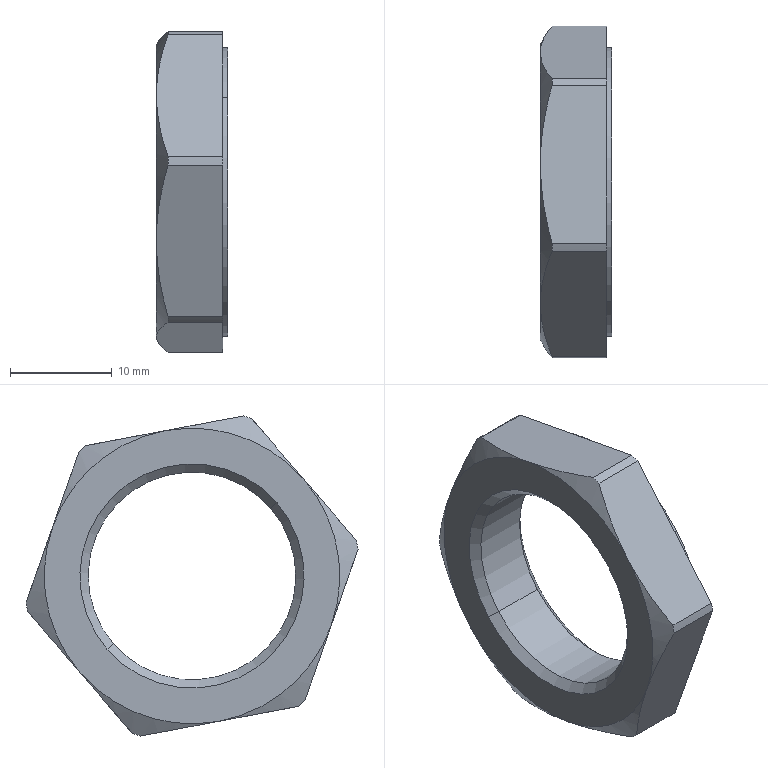Component | SolidWorks | CCDJSMA20x160SU(0)+(CS1-M-2)-1_CCDJS20 MA Nut-1 | 1 solid | 29 faces | box 7 x 32.58 x 31.42 mm | volume 2695 mm3 | cone 10 | cylinder 10 | plane 9 | commonest cylinder face diameters 33 x6 20.376 x2 28.4 x2
STEP:
#1=COLOUR_RGB('',0.7922,0.8196,0.9333);
#2=FILL_AREA_STYLE_COLOUR('',#1);
#3=FILL_AREA_STYLE('',(#2));
#4=SURFACE_STYLE_FILL_AREA(#3);
#5=SURFACE_SIDE_STYLE('',(#4));
#6=SURFACE_STYLE_USAGE(.BOTH.,#5);
#7=PRESENTATION_STYLE_ASSIGNMENT((#6));
#8=CARTESIAN_POINT('',(4.023,16.49,-2.241));
#9=VERTEX_POINT('',#8);
#10=CARTESIAN_POINT('',(4.023,17.098,-2.764));
#11=VERTEX_POINT('',#10);
#12=CARTESIAN_POINT('',(4.023,16.794,-2.503));
#13=DIRECTION('',(-1.,0.,0.));
#14=DIRECTION('',(0.,0.7584,-0.6518));
#15=AXIS2_PLACEMENT_3D('',#12,#13,#14);
#16=CIRCLE('',#15,0.4011);
#17=EDGE_CURVE('',#9,#11,#16,.T.);
#18=ORIENTED_EDGE('',*,*,#17,.T.);
#19=CARTESIAN_POINT('',(4.055,17.122,-2.785));
#20=VERTEX_POINT('',#19);
#21=CARTESIAN_POINT('',(4.055,17.122,-2.785));
#22=DIRECTION('',(0.7071,0.5363,-0.4609));
#23=VECTOR('',#22,39.37);
#24=LINE('',#21,#23);
#25=EDGE_CURVE('',#11,#20,#24,.T.);
#26=ORIENTED_EDGE('',*,*,#25,.T.);
#27=CARTESIAN_POINT('',(4.055,16.465,-2.22));
#28=VERTEX_POINT('',#27);
#29=CARTESIAN_POINT('',(4.055,16.794,-2.503));
#30=DIRECTION('',(-1.,0.,0.));
#31=DIRECTION('',(0.,0.7584,-0.6518));
#32=AXIS2_PLACEMENT_3D('',#29,#30,#31);
#33=CIRCLE('',#32,0.4331);
#34=EDGE_CURVE('',#28,#20,#33,.T.);
#35=ORIENTED_EDGE('',*,*,#34,.F.);
#36=CARTESIAN_POINT('',(4.055,16.465,-2.22));
#37=DIRECTION('',(0.7071,-0.5363,0.4609));
#38=VECTOR('',#37,39.37);
#39=LINE('',#36,#38);
#40=EDGE_CURVE('',#9,#28,#39,.T.);
#41=ORIENTED_EDGE('',*,*,#40,.F.);
#42=EDGE_LOOP('',(#18,#26,#35,#41));
#43=FACE_OUTER_BOUND('',#42,.T.);
#44=CARTESIAN_POINT('',(4.055,16.794,-2.503));
#45=DIRECTION('',(1.,0.,0.));
#46=DIRECTION('',(0.,-0.7584,0.6518));
#47=AXIS2_PLACEMENT_3D('',#44,#45,#46);
#48=CONICAL_SURFACE('',#47,0.4331,0.7854);
#49=ADVANCED_FACE('',(#43),#48,.F.);
#50=ORIENTED_EDGE('',*,*,#17,.F.);
#51=CARTESIAN_POINT('',(3.811,16.49,-2.241));
#52=VERTEX_POINT('',#51);
#53=CARTESIAN_POINT('',(4.055,16.49,-2.241));
#54=DIRECTION('',(-1.,0.,0.));
#55=VECTOR('',#54,39.37);
#56=LINE('',#53,#55);
#57=EDGE_CURVE('',#9,#52,#56,.T.);
#58=ORIENTED_EDGE('',*,*,#57,.T.);
#59=CARTESIAN_POINT('',(3.811,17.098,-2.764));
#60=VERTEX_POINT('',#59);
#61=CARTESIAN_POINT('',(3.811,16.794,-2.503));
#62=DIRECTION('',(-1.,0.,0.));
#63=DIRECTION('',(0.,0.7584,-0.6518));
#64=AXIS2_PLACEMENT_3D('',#61,#62,#63);
#65=CIRCLE('',#64,0.4011);
#66=EDGE_CURVE('',#52,#60,#65,.T.);
#67=ORIENTED_EDGE('',*,*,#66,.T.);
#68=CARTESIAN_POINT('',(4.055,17.098,-2.764));
#69=DIRECTION('',(-1.,0.,0.));
#70=VECTOR('',#69,39.37);
#71=LINE('',#68,#70);
#72=EDGE_CURVE('',#11,#60,#71,.T.);
#73=ORIENTED_EDGE('',*,*,#72,.F.);
#74=EDGE_LOOP('',(#50,#58,#67,#73));
#75=FACE_OUTER_BOUND('',#74,.T.);
#76=CARTESIAN_POINT('',(4.055,16.794,-2.503));
#77=DIRECTION('',(-1.,0.,0.));
#78=DIRECTION('',(0.,0.7584,-0.6518));
#79=AXIS2_PLACEMENT_3D('',#76,#77,#78);
#80=CYLINDRICAL_SURFACE('',#79,0.4011);
#81=ADVANCED_FACE('',(#75),#80,.F.);
#82=ORIENTED_EDGE('',*,*,#66,.F.);
#83=CARTESIAN_POINT('',(3.78,16.465,-2.22));
#84=VERTEX_POINT('',#83);
#85=CARTESIAN_POINT('',(3.811,16.49,-2.241));
#86=DIRECTION('',(-0.7071,-0.5363,0.4609));
#87=VECTOR('',#86,39.37);
#88=LINE('',#85,#87);
#89=EDGE_CURVE('',#52,#84,#88,.T.);
#90=ORIENTED_EDGE('',*,*,#89,.T.);
#91=CARTESIAN_POINT('',(3.78,17.122,-2.785));
#92=VERTEX_POINT('',#91);
#93=CARTESIAN_POINT('',(3.78,16.794,-2.503));
#94=DIRECTION('',(-1.,0.,0.));
#95=DIRECTION('',(0.,0.7584,-0.6518));
#96=AXIS2_PLACEMENT_3D('',#93,#94,#95);
#97=CIRCLE('',#96,0.4331);
#98=EDGE_CURVE('',#84,#92,#97,.T.);
#99=ORIENTED_EDGE('',*,*,#98,.T.);
#100=CARTESIAN_POINT('',(3.811,17.098,-2.764));
#101=DIRECTION('',(-0.7071,0.5363,-0.4609));
#102=VECTOR('',#101,39.37);
#103=LINE('',#100,#102);
#104=EDGE_CURVE('',#60,#92,#103,.T.);
#105=ORIENTED_EDGE('',*,*,#104,.F.);
#106=EDGE_LOOP('',(#82,#90,#99,#105));
#107=FACE_OUTER_BOUND('',#106,.T.);
#108=CARTESIAN_POINT('',(3.811,16.794,-2.503));
#109=DIRECTION('',(-1.,0.,0.));
#110=DIRECTION('',(0.,0.7584,-0.6518));
#111=AXIS2_PLACEMENT_3D('',#108,#109,#110);
#112=CONICAL_SURFACE('',#111,0.4011,0.7854);
#113=ADVANCED_FACE('',(#107),#112,.F.);
#114=CARTESIAN_POINT('',(4.055,17.218,-2.867));
#115=VERTEX_POINT('',#114);
#116=CARTESIAN_POINT('',(4.055,16.37,-2.138));
#117=VERTEX_POINT('',#116);
#118=CARTESIAN_POINT('',(4.055,16.794,-2.503));
#119=DIRECTION('',(-1.,0.,0.));
#120=DIRECTION('',(0.,0.7584,-0.6518));
#121=AXIS2_PLACEMENT_3D('',#118,#119,#120);
#122=CIRCLE('',#121,0.5591);
#123=EDGE_CURVE('',#115,#117,#122,.T.);
#124=ORIENTED_EDGE('',*,*,#123,.T.);
#125=CARTESIAN_POINT('',(4.035,16.37,-2.138));
#126=VERTEX_POINT('',#125);
#127=CARTESIAN_POINT('',(4.055,16.37,-2.138));
#128=DIRECTION('',(-1.,0.,0.));
#129=VECTOR('',#128,39.37);
#130=LINE('',#127,#129);
#131=EDGE_CURVE('',#117,#126,#130,.T.);
#132=ORIENTED_EDGE('',*,*,#131,.T.);
#133=CARTESIAN_POINT('',(4.035,17.218,-2.867));
#134=VERTEX_POINT('',#133);
#135=CARTESIAN_POINT('',(4.035,16.794,-2.503));
#136=DIRECTION('',(-1.,0.,0.));
#137=DIRECTION('',(0.,0.7584,-0.6518));
#138=AXIS2_PLACEMENT_3D('',#135,#136,#137);
#139=CIRCLE('',#138,0.5591);
#140=EDGE_CURVE('',#134,#126,#139,.T.);
#141=ORIENTED_EDGE('',*,*,#140,.F.);
#142=CARTESIAN_POINT('',(4.055,17.218,-2.867));
#143=DIRECTION('',(-1.,0.,0.));
#144=VECTOR('',#143,39.37);
#145=LINE('',#142,#144);
#146=EDGE_CURVE('',#115,#134,#145,.T.);
#147=ORIENTED_EDGE('',*,*,#146,.F.);
#148=EDGE_LOOP('',(#124,#132,#141,#147));
#149=FACE_OUTER_BOUND('',#148,.T.);
#150=CARTESIAN_POINT('',(4.055,16.794,-2.503));
#151=DIRECTION('',(-1.,0.,0.));
#152=DIRECTION('',(0.,0.7584,-0.6518));
#153=AXIS2_PLACEMENT_3D('',#150,#151,#152);
#154=CYLINDRICAL_SURFACE('',#153,0.5591);
#155=ADVANCED_FACE('',(#149),#154,.T.);
#156=CARTESIAN_POINT('',(3.825,17.435,-2.606));
#157=VERTEX_POINT('',#156);
#158=CARTESIAN_POINT('',(3.825,17.429,-2.64));
#159=VERTEX_POINT('',#158);
#160=CARTESIAN_POINT('',(3.825,16.794,-2.503));
#161=DIRECTION('',(-1.,0.,0.));
#162=DIRECTION('',(0.,0.7584,-0.6518));
#163=AXIS2_PLACEMENT_3D('',#160,#161,#162);
#164=CIRCLE('',#163,0.6496);
#165=EDGE_CURVE('',#157,#159,#164,.T.);
#166=ORIENTED_EDGE('',*,*,#165,.T.);
#167=CARTESIAN_POINT('',(3.78,17.227,-2.875));
#168=VERTEX_POINT('',#167);
#169=CARTESIAN_POINT('',(3.825,17.429,-2.64));
#170=CARTESIAN_POINT('',(3.811,17.396,-2.678));
#171=CARTESIAN_POINT('',(3.799,17.362,-2.717));
#172=CARTESIAN_POINT('',(3.784,17.295,-2.796));
#173=CARTESIAN_POINT('',(3.78,17.261,-2.835));
#174=CARTESIAN_POINT('',(3.78,17.227,-2.875));
#175=B_SPLINE_CURVE_WITH_KNOTS('',3,(#169,#170,#171,#172,#173,#174),.UNSPECIFIED.,.F.,.F.,(4,2,4),(0.01543,0.01941,0.02338),.UNSPECIFIED.);
#176=EDGE_CURVE('',#159,#168,#175,.T.);
#177=ORIENTED_EDGE('',*,*,#176,.T.);
#178=CARTESIAN_POINT('',(3.78,17.333,-2.314));
#179=VERTEX_POINT('',#178);
#180=CARTESIAN_POINT('',(3.78,16.794,-2.503));
#181=DIRECTION('',(-1.,0.,0.));
#182=DIRECTION('',(0.,0.7584,-0.6518));
#183=AXIS2_PLACEMENT_3D('',#180,#181,#182);
#184=CIRCLE('',#183,0.5709);
#185=EDGE_CURVE('',#179,#168,#184,.T.);
#186=ORIENTED_EDGE('',*,*,#185,.F.);
#187=CARTESIAN_POINT('',(3.78,17.333,-2.314));
#188=CARTESIAN_POINT('',(3.78,17.341,-2.339));
#189=CARTESIAN_POINT('',(3.781,17.35,-2.363));
#190=CARTESIAN_POINT('',(3.785,17.367,-2.413));
#191=CARTESIAN_POINT('',(3.788,17.376,-2.437));
#192=CARTESIAN_POINT('',(3.8,17.401,-2.51));
#193=CARTESIAN_POINT('',(3.811,17.418,-2.559));
#194=CARTESIAN_POINT('',(3.825,17.435,-2.606));
#195=B_SPLINE_CURVE_WITH_KNOTS('',3,(#187,#188,#189,#190,#191,#192,#193,#194),.UNSPECIFIED.,.F.,.F.,(4,2,2,4),(0.007958,0.009936,0.01191,0.01587),.UNSPECIFIED.);
#196=EDGE_CURVE('',#179,#157,#195,.T.);
#197=ORIENTED_EDGE('',*,*,#196,.T.);
#198=EDGE_LOOP('',(#166,#177,#186,#197));
#199=FACE_OUTER_BOUND('',#198,.T.);
#200=CARTESIAN_POINT('',(3.825,16.794,-2.503));
#201=DIRECTION('',(1.,0.,0.));
#202=DIRECTION('',(0.,-0.7584,0.6518));
#203=AXIS2_PLACEMENT_3D('',#200,#201,#202);
#204=CONICAL_SURFACE('',#203,0.6496,1.047);
#205=ADVANCED_FACE('',(#199),#204,.T.);
#206=CARTESIAN_POINT('',(3.825,17.204,-1.999));
#207=VERTEX_POINT('',#206);
#208=CARTESIAN_POINT('',(3.825,17.23,-2.021));
#209=VERTEX_POINT('',#208);
#210=CARTESIAN_POINT('',(3.825,16.794,-2.503));
#211=DIRECTION('',(-1.,0.,0.));
#212=DIRECTION('',(0.,0.7584,-0.6518));
#213=AXIS2_PLACEMENT_3D('',#210,#211,#212);
#214=CIRCLE('',#213,0.6496);
#215=EDGE_CURVE('',#207,#209,#214,.T.);
#216=ORIENTED_EDGE('',*,*,#215,.T.);
#217=CARTESIAN_POINT('',(3.825,17.23,-2.021));
#218=CARTESIAN_POINT('',(3.811,17.247,-2.069));
#219=CARTESIAN_POINT('',(3.8,17.264,-2.118));
#220=CARTESIAN_POINT('',(3.784,17.298,-2.215));
#221=CARTESIAN_POINT('',(3.78,17.315,-2.264));
#222=CARTESIAN_POINT('',(3.78,17.333,-2.314));
#223=B_SPLINE_CURVE_WITH_KNOTS('',3,(#217,#218,#219,#220,#221,#222),.UNSPECIFIED.,.F.,.F.,(4,2,4),(0.00000075,0.003979,0.007958),.UNSPECIFIED.);
#224=EDGE_CURVE('',#209,#179,#223,.T.);
#225=ORIENTED_EDGE('',*,*,#224,.T.);
#226=CARTESIAN_POINT('',(3.78,16.9,-1.942));
#227=VERTEX_POINT('',#226);
#228=CARTESIAN_POINT('',(3.78,16.794,-2.503));
#229=DIRECTION('',(-1.,0.,0.));
#230=DIRECTION('',(0.,0.7584,-0.6518));
#231=AXIS2_PLACEMENT_3D('',#228,#229,#230);
#232=CIRCLE('',#231,0.5709);
#233=EDGE_CURVE('',#227,#179,#232,.T.);
#234=ORIENTED_EDGE('',*,*,#233,.F.);
#235=CARTESIAN_POINT('',(3.78,16.9,-1.942));
#236=CARTESIAN_POINT('',(3.78,16.925,-1.947));
#237=CARTESIAN_POINT('',(3.781,16.951,-1.952));
#238=CARTESIAN_POINT('',(3.785,17.003,-1.961));
#239=CARTESIAN_POINT('',(3.788,17.028,-1.966));
#240=CARTESIAN_POINT('',(3.8,17.104,-1.98));
#241=CARTESIAN_POINT('',(3.811,17.155,-1.99));
#242=CARTESIAN_POINT('',(3.825,17.204,-1.999));
#243=B_SPLINE_CURVE_WITH_KNOTS('',3,(#235,#236,#237,#238,#239,#240,#241,#242),.UNSPECIFIED.,.F.,.F.,(4,2,2,4),(0.007958,0.009936,0.01191,0.01587),.UNSPECIFIED.);
#244=EDGE_CURVE('',#227,#207,#243,.T.);
#245=ORIENTED_EDGE('',*,*,#244,.T.);
#246=EDGE_LOOP('',(#216,#225,#234,#245));
#247=FACE_OUTER_BOUND('',#246,.T.);
#248=CARTESIAN_POINT('',(3.825,16.794,-2.503));
#249=DIRECTION('',(1.,0.,0.));
#250=DIRECTION('',(0.,-0.7584,0.6518));
#251=AXIS2_PLACEMENT_3D('',#248,#249,#250);
#252=CONICAL_SURFACE('',#251,0.6496,1.047);
#253=ADVANCED_FACE('',(#247),#252,.T.);
#254=CARTESIAN_POINT('',(3.825,16.563,-1.896));
#255=VERTEX_POINT('',#254);
#256=CARTESIAN_POINT('',(3.825,16.595,-1.884));
#257=VERTEX_POINT('',#256);
#258=CARTESIAN_POINT('',(3.825,16.794,-2.503));
#259=DIRECTION('',(-1.,0.,0.));
#260=DIRECTION('',(0.,0.7584,-0.6518));
#261=AXIS2_PLACEMENT_3D('',#258,#259,#260);
#262=CIRCLE('',#261,0.6496);
#263=EDGE_CURVE('',#255,#257,#262,.T.);
#264=ORIENTED_EDGE('',*,*,#263,.T.);
#265=CARTESIAN_POINT('',(3.825,16.595,-1.884));
#266=CARTESIAN_POINT('',(3.811,16.645,-1.894));
#267=CARTESIAN_POINT('',(3.8,16.695,-1.903));
#268=CARTESIAN_POINT('',(3.784,16.797,-1.922));
#269=CARTESIAN_POINT('',(3.78,16.848,-1.932));
#270=CARTESIAN_POINT('',(3.78,16.9,-1.942));
#271=B_SPLINE_CURVE_WITH_KNOTS('',3,(#265,#266,#267,#268,#269,#270),.UNSPECIFIED.,.F.,.F.,(4,2,4),(0.00000075,0.003979,0.007958),.UNSPECIFIED.);
#272=EDGE_CURVE('',#257,#227,#271,.T.);
#273=ORIENTED_EDGE('',*,*,#272,.T.);
#274=CARTESIAN_POINT('',(3.78,16.361,-2.131));
#275=VERTEX_POINT('',#274);
#276=CARTESIAN_POINT('',(3.78,16.794,-2.503));
#277=DIRECTION('',(-1.,0.,0.));
#278=DIRECTION('',(0.,0.7584,-0.6518));
#279=AXIS2_PLACEMENT_3D('',#276,#277,#278);
#280=CIRCLE('',#279,0.5709);
#281=EDGE_CURVE('',#275,#227,#280,.T.);
#282=ORIENTED_EDGE('',*,*,#281,.F.);
#283=CARTESIAN_POINT('',(3.78,16.361,-2.131));
#284=CARTESIAN_POINT('',(3.78,16.395,-2.091));
#285=CARTESIAN_POINT('',(3.784,16.429,-2.052));
#286=CARTESIAN_POINT('',(3.799,16.496,-1.973));
#287=CARTESIAN_POINT('',(3.811,16.53,-1.934));
#288=CARTESIAN_POINT('',(3.825,16.563,-1.896));
#289=B_SPLINE_CURVE_WITH_KNOTS('',3,(#283,#284,#285,#286,#287,#288),.UNSPECIFIED.,.F.,.F.,(4,2,4),(0.01461,0.01858,0.02255),.UNSPECIFIED.);
#290=EDGE_CURVE('',#275,#255,#289,.T.);
#291=ORIENTED_EDGE('',*,*,#290,.T.);
#292=EDGE_LOOP('',(#264,#273,#282,#291));
#293=FACE_OUTER_BOUND('',#292,.T.);
#294=CARTESIAN_POINT('',(3.825,16.794,-2.503));
#295=DIRECTION('',(1.,0.,0.));
#296=DIRECTION('',(0.,-0.7584,0.6518));
#297=AXIS2_PLACEMENT_3D('',#294,#295,#296);
#298=CONICAL_SURFACE('',#297,0.6496,1.047);
#299=ADVANCED_FACE('',(#293),#298,.T.);
#300=CARTESIAN_POINT('',(3.825,16.153,-2.399));
#301=VERTEX_POINT('',#300);
#302=CARTESIAN_POINT('',(3.825,16.159,-2.366));
#303=VERTEX_POINT('',#302);
#304=CARTESIAN_POINT('',(3.825,16.794,-2.503));
#305=DIRECTION('',(-1.,0.,0.));
#306=DIRECTION('',(0.,0.7584,-0.6518));
#307=AXIS2_PLACEMENT_3D('',#304,#305,#306);
#308=CIRCLE('',#307,0.6496);
#309=EDGE_CURVE('',#301,#303,#308,.T.);
#310=ORIENTED_EDGE('',*,*,#309,.T.);
#311=CARTESIAN_POINT('',(3.825,16.159,-2.366));
#312=CARTESIAN_POINT('',(3.811,16.192,-2.328));
#313=CARTESIAN_POINT('',(3.8,16.225,-2.289));
#314=CARTESIAN_POINT('',(3.788,16.275,-2.23));
#315=CARTESIAN_POINT('',(3.785,16.292,-2.21));
#316=CARTESIAN_POINT('',(3.781,16.327,-2.17));
#317=CARTESIAN_POINT('',(3.78,16.344,-2.151));
#318=CARTESIAN_POINT('',(3.78,16.361,-2.131));
#319=B_SPLINE_CURVE_WITH_KNOTS('',3,(#311,#312,#313,#314,#315,#316,#317,#318),.UNSPECIFIED.,.F.,.F.,(4,2,2,4),(0.006677,0.01064,0.01263,0.01461),.UNSPECIFIED.);
#320=EDGE_CURVE('',#303,#275,#319,.T.);
#321=ORIENTED_EDGE('',*,*,#320,.T.);
#322=CARTESIAN_POINT('',(3.78,16.255,-2.692));
#323=VERTEX_POINT('',#322);
#324=CARTESIAN_POINT('',(3.78,16.794,-2.503));
#325=DIRECTION('',(-1.,0.,0.));
#326=DIRECTION('',(0.,0.7584,-0.6518));
#327=AXIS2_PLACEMENT_3D('',#324,#325,#326);
#328=CIRCLE('',#327,0.5709);
#329=EDGE_CURVE('',#323,#275,#328,.T.);
#330=ORIENTED_EDGE('',*,*,#329,.F.);
#331=CARTESIAN_POINT('',(3.78,16.255,-2.692));
#332=CARTESIAN_POINT('',(3.78,16.247,-2.667));
#333=CARTESIAN_POINT('',(3.781,16.238,-2.642));
#334=CARTESIAN_POINT('',(3.785,16.22,-2.593));
#335=CARTESIAN_POINT('',(3.788,16.212,-2.568));
#336=CARTESIAN_POINT('',(3.8,16.186,-2.495));
#337=CARTESIAN_POINT('',(3.811,16.169,-2.447));
#338=CARTESIAN_POINT('',(3.825,16.153,-2.399));
#339=B_SPLINE_CURVE_WITH_KNOTS('',3,(#331,#332,#333,#334,#335,#336,#337,#338),.UNSPECIFIED.,.F.,.F.,(4,2,2,4),(0.007958,0.009936,0.01191,0.01587),.UNSPECIFIED.);
#340=EDGE_CURVE('',#323,#301,#339,.T.);
#341=ORIENTED_EDGE('',*,*,#340,.T.);
#342=EDGE_LOOP('',(#310,#321,#330,#341));
#343=FACE_OUTER_BOUND('',#342,.T.);
#344=CARTESIAN_POINT('',(3.825,16.794,-2.503));
#345=DIRECTION('',(1.,0.,0.));
#346=DIRECTION('',(0.,-0.7584,0.6518));
#347=AXIS2_PLACEMENT_3D('',#344,#345,#346);
#348=CONICAL_SURFACE('',#347,0.6496,1.047);
#349=ADVANCED_FACE('',(#343),#348,.T.);
#350=CARTESIAN_POINT('',(3.825,16.383,-3.006));
#351=VERTEX_POINT('',#350);
#352=CARTESIAN_POINT('',(3.825,16.358,-2.984));
#353=VERTEX_POINT('',#352);
#354=CARTESIAN_POINT('',(3.825,16.794,-2.503));
#355=DIRECTION('',(-1.,0.,0.));
#356=DIRECTION('',(0.,0.7584,-0.6518));
#357=AXIS2_PLACEMENT_3D('',#354,#355,#356);
#358=CIRCLE('',#357,0.6496);
#359=EDGE_CURVE('',#351,#353,#358,.T.);
#360=ORIENTED_EDGE('',*,*,#359,.T.);
#361=CARTESIAN_POINT('',(3.825,16.358,-2.984));
#362=CARTESIAN_POINT('',(3.811,16.341,-2.936));
#363=CARTESIAN_POINT('',(3.8,16.324,-2.888));
#364=CARTESIAN_POINT('',(3.784,16.29,-2.79));
#365=CARTESIAN_POINT('',(3.78,16.273,-2.741));
#366=CARTESIAN_POINT('',(3.78,16.255,-2.692));
#367=B_SPLINE_CURVE_WITH_KNOTS('',3,(#361,#362,#363,#364,#365,#366),.UNSPECIFIED.,.F.,.F.,(4,2,4),(0.00000075,0.003979,0.007958),.UNSPECIFIED.);
#368=EDGE_CURVE('',#353,#323,#367,.T.);
#369=ORIENTED_EDGE('',*,*,#368,.T.);
#370=CARTESIAN_POINT('',(3.78,16.688,-3.064));
#371=VERTEX_POINT('',#370);
#372=CARTESIAN_POINT('',(3.78,16.794,-2.503));
#373=DIRECTION('',(-1.,0.,0.));
#374=DIRECTION('',(0.,0.7584,-0.6518));
#375=AXIS2_PLACEMENT_3D('',#372,#373,#374);
#376=CIRCLE('',#375,0.5709);
#377=EDGE_CURVE('',#371,#323,#376,.T.);
#378=ORIENTED_EDGE('',*,*,#377,.F.);
#379=CARTESIAN_POINT('',(3.78,16.688,-3.064));
#380=CARTESIAN_POINT('',(3.78,16.662,-3.059));
#381=CARTESIAN_POINT('',(3.781,16.636,-3.054));
#382=CARTESIAN_POINT('',(3.785,16.585,-3.044));
#383=CARTESIAN_POINT('',(3.788,16.56,-3.04));
#384=CARTESIAN_POINT('',(3.8,16.483,-3.025));
#385=CARTESIAN_POINT('',(3.811,16.433,-3.016));
#386=CARTESIAN_POINT('',(3.825,16.383,-3.006));
#387=B_SPLINE_CURVE_WITH_KNOTS('',3,(#379,#380,#381,#382,#383,#384,#385,#386),.UNSPECIFIED.,.F.,.F.,(4,2,2,4),(0.007958,0.009936,0.01191,0.01587),.UNSPECIFIED.);
#388=EDGE_CURVE('',#371,#351,#387,.T.);
#389=ORIENTED_EDGE('',*,*,#388,.T.);
#390=EDGE_LOOP('',(#360,#369,#378,#389));
#391=FACE_OUTER_BOUND('',#390,.T.);
#392=CARTESIAN_POINT('',(3.825,16.794,-2.503));
#393=DIRECTION('',(1.,0.,0.));
#394=DIRECTION('',(0.,-0.7584,0.6518));
#395=AXIS2_PLACEMENT_3D('',#392,#393,#394);
#396=CONICAL_SURFACE('',#395,0.6496,1.047);
#397=ADVANCED_FACE('',(#391),#396,.T.);
#398=CARTESIAN_POINT('',(4.035,17.435,-2.606));
#399=VERTEX_POINT('',#398);
#400=CARTESIAN_POINT('',(4.035,17.429,-2.64));
#401=VERTEX_POINT('',#400);
#402=CARTESIAN_POINT('',(4.035,16.794,-2.503));
#403=DIRECTION('',(-1.,0.,0.));
#404=DIRECTION('',(0.,0.7584,-0.6518));
#405=AXIS2_PLACEMENT_3D('',#402,#403,#404);
#406=CIRCLE('',#405,0.6496);
#407=EDGE_CURVE('',#399,#401,#406,.T.);
#408=ORIENTED_EDGE('',*,*,#407,.T.);
#409=CARTESIAN_POINT('',(4.055,17.429,-2.64));
#410=DIRECTION('',(-1.,0.,0.));
#411=VECTOR('',#410,39.37);
#412=LINE('',#409,#411);
#413=EDGE_CURVE('',#401,#159,#412,.T.);
#414=ORIENTED_EDGE('',*,*,#413,.T.);
#415=ORIENTED_EDGE('',*,*,#165,.F.);
#416=CARTESIAN_POINT('',(4.055,17.435,-2.606));
#417=DIRECTION('',(1.,0.,0.));
#418=VECTOR('',#417,39.37);
#419=LINE('',#416,#418);
#420=EDGE_CURVE('',#157,#399,#419,.T.);
#421=ORIENTED_EDGE('',*,*,#420,.T.);
#422=EDGE_LOOP('',(#408,#414,#415,#421));
#423=FACE_OUTER_BOUND('',#422,.T.);
#424=CARTESIAN_POINT('',(4.055,16.794,-2.503));
#425=DIRECTION('',(-1.,0.,0.));
#426=DIRECTION('',(0.,0.7584,-0.6518));
#427=AXIS2_PLACEMENT_3D('',#424,#425,#426);
#428=CYLINDRICAL_SURFACE('',#427,0.6496);
#429=ADVANCED_FACE('',(#423),#428,.T.);
#430=CARTESIAN_POINT('',(4.035,17.204,-1.999));
#431=VERTEX_POINT('',#430);
#432=CARTESIAN_POINT('',(4.035,17.23,-2.021));
#433=VERTEX_POINT('',#432);
#434=CARTESIAN_POINT('',(4.035,16.794,-2.503));
#435=DIRECTION('',(-1.,0.,0.));
#436=DIRECTION('',(0.,0.7584,-0.6518));
#437=AXIS2_PLACEMENT_3D('',#434,#435,#436);
#438=CIRCLE('',#437,0.6496);
#439=EDGE_CURVE('',#431,#433,#438,.T.);
#440=ORIENTED_EDGE('',*,*,#439,.T.);
#441=CARTESIAN_POINT('',(4.055,17.23,-2.021));
#442=DIRECTION('',(-1.,0.,0.));
#443=VECTOR('',#442,39.37);
#444=LINE('',#441,#443);
#445=EDGE_CURVE('',#433,#209,#444,.T.);
#446=ORIENTED_EDGE('',*,*,#445,.T.);
#447=ORIENTED_EDGE('',*,*,#215,.F.);
#448=CARTESIAN_POINT('',(4.055,17.204,-1.999));
#449=DIRECTION('',(1.,0.,0.));
#450=VECTOR('',#449,39.37);
#451=LINE('',#448,#450);
#452=EDGE_CURVE('',#207,#431,#451,.T.);
#453=ORIENTED_EDGE('',*,*,#452,.T.);
#454=EDGE_LOOP('',(#440,#446,#447,#453));
#455=FACE_OUTER_BOUND('',#454,.T.);
#456=CARTESIAN_POINT('',(4.055,16.794,-2.503));
#457=DIRECTION('',(-1.,0.,0.));
#458=DIRECTION('',(0.,0.7584,-0.6518));
#459=AXIS2_PLACEMENT_3D('',#456,#457,#458);
#460=CYLINDRICAL_SURFACE('',#459,0.6496);
#461=ADVANCED_FACE('',(#455),#460,.T.);
#462=CARTESIAN_POINT('',(4.035,16.563,-1.896));
#463=VERTEX_POINT('',#462);
#464=CARTESIAN_POINT('',(4.035,16.595,-1.884));
#465=VERTEX_POINT('',#464);
#466=CARTESIAN_POINT('',(4.035,16.794,-2.503));
#467=DIRECTION('',(-1.,0.,0.));
#468=DIRECTION('',(0.,0.7584,-0.6518));
#469=AXIS2_PLACEMENT_3D('',#466,#467,#468);
#470=CIRCLE('',#469,0.6496);
#471=EDGE_CURVE('',#463,#465,#470,.T.);
#472=ORIENTED_EDGE('',*,*,#471,.T.);
#473=CARTESIAN_POINT('',(4.055,16.595,-1.884));
#474=DIRECTION('',(-1.,0.,0.));
#475=VECTOR('',#474,39.37);
#476=LINE('',#473,#475);
#477=EDGE_CURVE('',#465,#257,#476,.T.);
#478=ORIENTED_EDGE('',*,*,#477,.T.);
#479=ORIENTED_EDGE('',*,*,#263,.F.);
#480=CARTESIAN_POINT('',(4.055,16.563,-1.896));
#481=DIRECTION('',(1.,0.,0.));
#482=VECTOR('',#481,39.37);
#483=LINE('',#480,#482);
#484=EDGE_CURVE('',#255,#463,#483,.T.);
#485=ORIENTED_EDGE('',*,*,#484,.T.);
#486=EDGE_LOOP('',(#472,#478,#479,#485));
#487=FACE_OUTER_BOUND('',#486,.T.);
#488=CARTESIAN_POINT('',(4.055,16.794,-2.503));
#489=DIRECTION('',(-1.,0.,0.));
#490=DIRECTION('',(0.,0.7584,-0.6518));
#491=AXIS2_PLACEMENT_3D('',#488,#489,#490);
#492=CYLINDRICAL_SURFACE('',#491,0.6496);
#493=ADVANCED_FACE('',(#487),#492,.T.);
#494=CARTESIAN_POINT('',(4.035,16.153,-2.399));
#495=VERTEX_POINT('',#494);
#496=CARTESIAN_POINT('',(4.035,16.159,-2.366));
#497=VERTEX_POINT('',#496);
#498=CARTESIAN_POINT('',(4.035,16.794,-2.503));
#499=DIRECTION('',(-1.,0.,0.));
#500=DIRECTION('',(0.,0.7584,-0.6518));
#501=AXIS2_PLACEMENT_3D('',#498,#499,#500);
#502=CIRCLE('',#501,0.6496);
#503=EDGE_CURVE('',#495,#497,#502,.T.);
#504=ORIENTED_EDGE('',*,*,#503,.T.);
#505=CARTESIAN_POINT('',(4.055,16.159,-2.366));
#506=DIRECTION('',(-1.,0.,0.));
#507=VECTOR('',#506,39.37);
#508=LINE('',#505,#507);
#509=EDGE_CURVE('',#497,#303,#508,.T.);
#510=ORIENTED_EDGE('',*,*,#509,.T.);
#511=ORIENTED_EDGE('',*,*,#309,.F.);
#512=CARTESIAN_POINT('',(4.055,16.153,-2.399));
#513=DIRECTION('',(1.,0.,0.));
#514=VECTOR('',#513,39.37);
#515=LINE('',#512,#514);
#516=EDGE_CURVE('',#301,#495,#515,.T.);
#517=ORIENTED_EDGE('',*,*,#516,.T.);
#518=EDGE_LOOP('',(#504,#510,#511,#517));
#519=FACE_OUTER_BOUND('',#518,.T.);
#520=CARTESIAN_POINT('',(4.055,16.794,-2.503));
#521=DIRECTION('',(-1.,0.,0.));
#522=DIRECTION('',(0.,0.7584,-0.6518));
#523=AXIS2_PLACEMENT_3D('',#520,#521,#522);
#524=CYLINDRICAL_SURFACE('',#523,0.6496);
#525=ADVANCED_FACE('',(#519),#524,.T.);
#526=CARTESIAN_POINT('',(4.035,16.383,-3.006));
#527=VERTEX_POINT('',#526);
#528=CARTESIAN_POINT('',(4.035,16.358,-2.984));
#529=VERTEX_POINT('',#528);
#530=CARTESIAN_POINT('',(4.035,16.794,-2.503));
#531=DIRECTION('',(-1.,0.,0.));
#532=DIRECTION('',(0.,0.7584,-0.6518));
#533=AXIS2_PLACEMENT_3D('',#530,#531,#532);
#534=CIRCLE('',#533,0.6496);
#535=EDGE_CURVE('',#527,#529,#534,.T.);
#536=ORIENTED_EDGE('',*,*,#535,.T.);
#537=CARTESIAN_POINT('',(4.055,16.358,-2.984));
#538=DIRECTION('',(-1.,0.,0.));
#539=VECTOR('',#538,39.37);
#540=LINE('',#537,#539);
#541=EDGE_CURVE('',#529,#353,#540,.T.);
#542=ORIENTED_EDGE('',*,*,#541,.T.);
#543=ORIENTED_EDGE('',*,*,#359,.F.);
#544=CARTESIAN_POINT('',(4.055,16.383,-3.006));
#545=DIRECTION('',(1.,0.,0.));
#546=VECTOR('',#545,39.37);
#547=LINE('',#544,#546);
#548=EDGE_CURVE('',#351,#527,#547,.T.);
#549=ORIENTED_EDGE('',*,*,#548,.T.);
#550=EDGE_LOOP('',(#536,#542,#543,#549));
#551=FACE_OUTER_BOUND('',#550,.T.);
#552=CARTESIAN_POINT('',(4.055,16.794,-2.503));
#553=DIRECTION('',(-1.,0.,0.));
#554=DIRECTION('',(0.,0.7584,-0.6518));
#555=AXIS2_PLACEMENT_3D('',#552,#553,#554);
#556=CYLINDRICAL_SURFACE('',#555,0.6496);
#557=ADVANCED_FACE('',(#551),#556,.T.);
#558=CARTESIAN_POINT('',(3.78,16.794,-2.503));
#559=DIRECTION('',(-1.,0.,0.));
#560=DIRECTION('',(0.,0.7584,-0.6518));
#561=AXIS2_PLACEMENT_3D('',#558,#559,#560);
#562=CIRCLE('',#561,0.4331);
#563=EDGE_CURVE('',#92,#84,#562,.T.);
#564=ORIENTED_EDGE('',*,*,#563,.F.);
#565=ORIENTED_EDGE('',*,*,#98,.F.);
#566=EDGE_LOOP('',(#564,#565));
#567=FACE_BOUND('',#566,.T.);
#568=CARTESIAN_POINT('',(3.78,16.794,-2.503));
#569=DIRECTION('',(-1.,0.,0.));
#570=DIRECTION('',(0.,0.7584,-0.6518));
#571=AXIS2_PLACEMENT_3D('',#568,#569,#570);
#572=CIRCLE('',#571,0.5709);
#573=EDGE_CURVE('',#168,#371,#572,.T.);
#574=ORIENTED_EDGE('',*,*,#573,.T.);
#575=ORIENTED_EDGE('',*,*,#377,.T.);
#576=ORIENTED_EDGE('',*,*,#329,.T.);
#577=ORIENTED_EDGE('',*,*,#281,.T.);
#578=ORIENTED_EDGE('',*,*,#233,.T.);
#579=ORIENTED_EDGE('',*,*,#185,.T.);
#580=EDGE_LOOP('',(#574,#575,#576,#577,#578,#579));
#581=FACE_OUTER_BOUND('',#580,.T.);
#582=CARTESIAN_POINT('',(3.78,16.794,-2.503));
#583=DIRECTION('',(1.,0.,0.));
#584=DIRECTION('',(0.,-0.7584,0.6518));
#585=AXIS2_PLACEMENT_3D('',#582,#583,#584);
#586=PLANE('',#585);
#587=ADVANCED_FACE('',(#567,#581),#586,.F.);
#588=ORIENTED_EDGE('',*,*,#573,.F.);
#589=CARTESIAN_POINT('',(3.825,17.025,-3.11));
#590=VERTEX_POINT('',#589);
#591=CARTESIAN_POINT('',(3.78,17.227,-2.875));
#592=CARTESIAN_POINT('',(3.78,17.21,-2.895));
#593=CARTESIAN_POINT('',(3.781,17.193,-2.915));
#594=CARTESIAN_POINT('',(3.785,17.158,-2.954));
#595=CARTESIAN_POINT('',(3.788,17.141,-2.974));
#596=CARTESIAN_POINT('',(3.8,17.091,-3.033));
#597=CARTESIAN_POINT('',(3.811,17.057,-3.072));
#598=CARTESIAN_POINT('',(3.825,17.025,-3.11));
#599=B_SPLINE_CURVE_WITH_KNOTS('',3,(#591,#592,#593,#594,#595,#596,#597,#598),.UNSPECIFIED.,.F.,.F.,(4,2,2,4),(0.02338,0.02537,0.02736,0.03134),.UNSPECIFIED.);
#600=EDGE_CURVE('',#168,#590,#599,.T.);
#601=ORIENTED_EDGE('',*,*,#600,.T.);
#602=CARTESIAN_POINT('',(3.825,16.993,-3.121));
#603=VERTEX_POINT('',#602);
#604=CARTESIAN_POINT('',(3.825,16.794,-2.503));
#605=DIRECTION('',(-1.,0.,0.));
#606=DIRECTION('',(0.,0.7584,-0.6518));
#607=AXIS2_PLACEMENT_3D('',#604,#605,#606);
#608=CIRCLE('',#607,0.6496);
#609=EDGE_CURVE('',#590,#603,#608,.T.);
#610=ORIENTED_EDGE('',*,*,#609,.T.);
#611=CARTESIAN_POINT('',(3.825,16.993,-3.121));
#612=CARTESIAN_POINT('',(3.811,16.943,-3.112));
#613=CARTESIAN_POINT('',(3.8,16.892,-3.102));
#614=CARTESIAN_POINT('',(3.784,16.791,-3.083));
#615=CARTESIAN_POINT('',(3.78,16.74,-3.073));
#616=CARTESIAN_POINT('',(3.78,16.688,-3.064));
#617=B_SPLINE_CURVE_WITH_KNOTS('',3,(#611,#612,#613,#614,#615,#616),.UNSPECIFIED.,.F.,.F.,(4,2,4),(0.00000075,0.003979,0.007958),.UNSPECIFIED.);
#618=EDGE_CURVE('',#603,#371,#617,.T.);
#619=ORIENTED_EDGE('',*,*,#618,.T.);
#620=EDGE_LOOP('',(#588,#601,#610,#619));
#621=FACE_OUTER_BOUND('',#620,.T.);
#622=CARTESIAN_POINT('',(3.825,16.794,-2.503));
#623=DIRECTION('',(1.,0.,0.));
#624=DIRECTION('',(0.,-0.7584,0.6518));
#625=AXIS2_PLACEMENT_3D('',#622,#623,#624);
#626=CONICAL_SURFACE('',#625,0.6496,1.047);
#627=ADVANCED_FACE('',(#621),#626,.T.);
#628=ORIENTED_EDGE('',*,*,#609,.F.);
#629=CARTESIAN_POINT('',(4.035,17.025,-3.11));
#630=VERTEX_POINT('',#629);
#631=CARTESIAN_POINT('',(4.055,17.025,-3.11));
#632=DIRECTION('',(1.,0.,0.));
#633=VECTOR('',#632,39.37);
#634=LINE('',#631,#633);
#635=EDGE_CURVE('',#590,#630,#634,.T.);
#636=ORIENTED_EDGE('',*,*,#635,.T.);
#637=CARTESIAN_POINT('',(4.035,16.993,-3.121));
#638=VERTEX_POINT('',#637);
#639=CARTESIAN_POINT('',(4.035,16.794,-2.503));
#640=DIRECTION('',(-1.,0.,0.));
#641=DIRECTION('',(0.,0.7584,-0.6518));
#642=AXIS2_PLACEMENT_3D('',#639,#640,#641);
#643=CIRCLE('',#642,0.6496);
#644=EDGE_CURVE('',#630,#638,#643,.T.);
#645=ORIENTED_EDGE('',*,*,#644,.T.);
#646=CARTESIAN_POINT('',(4.055,16.993,-3.121));
#647=DIRECTION('',(-1.,0.,0.));
#648=VECTOR('',#647,39.37);
#649=LINE('',#646,#648);
#650=EDGE_CURVE('',#638,#603,#649,.T.);
#651=ORIENTED_EDGE('',*,*,#650,.T.);
#652=EDGE_LOOP('',(#628,#636,#645,#651));
#653=FACE_OUTER_BOUND('',#652,.T.);
#654=CARTESIAN_POINT('',(4.055,16.794,-2.503));
#655=DIRECTION('',(-1.,0.,0.));
#656=DIRECTION('',(0.,0.7584,-0.6518));
#657=AXIS2_PLACEMENT_3D('',#654,#655,#656);
#658=CYLINDRICAL_SURFACE('',#657,0.6496);
#659=ADVANCED_FACE('',(#653),#658,.T.);
#660=ORIENTED_EDGE('',*,*,#644,.F.);
#661=CARTESIAN_POINT('',(4.035,16.803,-3.368));
#662=DIRECTION('',(0.,0.6518,0.7584));
#663=VECTOR('',#662,39.37);
#664=LINE('',#661,#663);
#665=EDGE_CURVE('',#630,#401,#664,.T.);
#666=ORIENTED_EDGE('',*,*,#665,.T.);
#667=ORIENTED_EDGE('',*,*,#407,.F.);
#668=CARTESIAN_POINT('',(4.035,17.44,-2.62));
#669=DIRECTION('',(0.,-0.3309,0.9437));
#670=VECTOR('',#669,39.37);
#671=LINE('',#668,#670);
#672=EDGE_CURVE('',#399,#433,#671,.T.);
#673=ORIENTED_EDGE('',*,*,#672,.T.);
#674=ORIENTED_EDGE('',*,*,#439,.F.);
#675=CARTESIAN_POINT('',(4.035,16.58,-1.882));
#676=DIRECTION('',(0.,-0.9827,0.1853));
#677=VECTOR('',#676,39.37);
#678=LINE('',#675,#677);
#679=EDGE_CURVE('',#431,#465,#678,.T.);
#680=ORIENTED_EDGE('',*,*,#679,.T.);
#681=ORIENTED_EDGE('',*,*,#471,.F.);
#682=CARTESIAN_POINT('',(4.035,15.938,-2.623));
#683=DIRECTION('',(0.,-0.6518,-0.7584));
#684=VECTOR('',#683,39.37);
#685=LINE('',#682,#684);
#686=EDGE_CURVE('',#463,#497,#685,.T.);
#687=ORIENTED_EDGE('',*,*,#686,.T.);
#688=ORIENTED_EDGE('',*,*,#503,.F.);
#689=CARTESIAN_POINT('',(4.035,16.363,-2.998));
#690=DIRECTION('',(0.,0.3309,-0.9437));
#691=VECTOR('',#690,39.37);
#692=LINE('',#689,#691);
#693=EDGE_CURVE('',#495,#529,#692,.T.);
#694=ORIENTED_EDGE('',*,*,#693,.T.);
#695=ORIENTED_EDGE('',*,*,#535,.F.);
#696=CARTESIAN_POINT('',(4.035,16.369,-3.004));
#697=DIRECTION('',(0.,0.9827,-0.1853));
#698=VECTOR('',#697,39.37);
#699=LINE('',#696,#698);
#700=EDGE_CURVE('',#527,#638,#699,.T.);
#701=ORIENTED_EDGE('',*,*,#700,.T.);
#702=EDGE_LOOP('',(#660,#666,#667,#673,#674,#680,#681,#687,#688,#694,#695,#701));
#703=FACE_OUTER_BOUND('',#702,.T.);
#704=ORIENTED_EDGE('',*,*,#140,.T.);
#705=CARTESIAN_POINT('',(4.035,16.794,-2.503));
#706=DIRECTION('',(-1.,0.,0.));
#707=DIRECTION('',(0.,0.7584,-0.6518));
#708=AXIS2_PLACEMENT_3D('',#705,#706,#707);
#709=CIRCLE('',#708,0.5591);
#710=EDGE_CURVE('',#126,#134,#709,.T.);
#711=ORIENTED_EDGE('',*,*,#710,.T.);
#712=EDGE_LOOP('',(#704,#711));
#713=FACE_BOUND('',#712,.T.);
#714=CARTESIAN_POINT('',(4.035,16.37,-2.995));
#715=DIRECTION('',(-1.,0.,0.));
#716=DIRECTION('',(0.,0.7584,-0.6518));
#717=AXIS2_PLACEMENT_3D('',#714,#715,#716);
#718=PLANE('',#717);
#719=ADVANCED_FACE('',(#703,#713),#718,.F.);
#720=ORIENTED_EDGE('',*,*,#131,.F.);
#721=CARTESIAN_POINT('',(4.055,16.794,-2.503));
#722=DIRECTION('',(-1.,0.,0.));
#723=DIRECTION('',(0.,0.7584,-0.6518));
#724=AXIS2_PLACEMENT_3D('',#721,#722,#723);
#725=CIRCLE('',#724,0.5591);
#726=EDGE_CURVE('',#117,#115,#725,.T.);
#727=ORIENTED_EDGE('',*,*,#726,.T.);
#728=ORIENTED_EDGE('',*,*,#146,.T.);
#729=ORIENTED_EDGE('',*,*,#710,.F.);
#730=EDGE_LOOP('',(#720,#727,#728,#729));
#731=FACE_OUTER_BOUND('',#730,.T.);
#732=CARTESIAN_POINT('',(4.055,16.794,-2.503));
#733=DIRECTION('',(-1.,0.,0.));
#734=DIRECTION('',(0.,0.7584,-0.6518));
#735=AXIS2_PLACEMENT_3D('',#732,#733,#734);
#736=CYLINDRICAL_SURFACE('',#735,0.5591);
#737=ADVANCED_FACE('',(#731),#736,.T.);
#738=ORIENTED_EDGE('',*,*,#34,.T.);
#739=CARTESIAN_POINT('',(4.055,16.794,-2.503));
#740=DIRECTION('',(-1.,0.,0.));
#741=DIRECTION('',(0.,0.7584,-0.6518));
#742=AXIS2_PLACEMENT_3D('',#739,#740,#741);
#743=CIRCLE('',#742,0.4331);
#744=EDGE_CURVE('',#20,#28,#743,.T.);
#745=ORIENTED_EDGE('',*,*,#744,.T.);
#746=EDGE_LOOP('',(#738,#745));
#747=FACE_BOUND('',#746,.T.);
#748=ORIENTED_EDGE('',*,*,#123,.F.);
#749=ORIENTED_EDGE('',*,*,#726,.F.);
#750=EDGE_LOOP('',(#748,#749));
#751=FACE_OUTER_BOUND('',#750,.T.);
#752=CARTESIAN_POINT('',(4.055,16.429,-2.927));
#753=DIRECTION('',(-1.,0.,0.));
#754=DIRECTION('',(0.,0.7584,-0.6518));
#755=AXIS2_PLACEMENT_3D('',#752,#753,#754);
#756=PLANE('',#755);
#757=ADVANCED_FACE('',(#747,#751),#756,.F.);
#758=ORIENTED_EDGE('',*,*,#89,.F.);
#759=CARTESIAN_POINT('',(3.811,16.794,-2.503));
#760=DIRECTION('',(-1.,0.,0.));
#761=DIRECTION('',(0.,0.7584,-0.6518));
#762=AXIS2_PLACEMENT_3D('',#759,#760,#761);
#763=CIRCLE('',#762,0.4011);
#764=EDGE_CURVE('',#60,#52,#763,.T.);
#765=ORIENTED_EDGE('',*,*,#764,.F.);
#766=ORIENTED_EDGE('',*,*,#104,.T.);
#767=ORIENTED_EDGE('',*,*,#563,.T.);
#768=EDGE_LOOP('',(#758,#765,#766,#767));
#769=FACE_OUTER_BOUND('',#768,.T.);
#770=CARTESIAN_POINT('',(3.811,16.794,-2.503));
#771=DIRECTION('',(-1.,0.,0.));
#772=DIRECTION('',(0.,0.7584,-0.6518));
#773=AXIS2_PLACEMENT_3D('',#770,#771,#772);
#774=CONICAL_SURFACE('',#773,0.4011,0.7854);
#775=ADVANCED_FACE('',(#769),#774,.F.);
#776=ORIENTED_EDGE('',*,*,#57,.F.);
#777=CARTESIAN_POINT('',(4.023,16.794,-2.503));
#778=DIRECTION('',(-1.,0.,0.));
#779=DIRECTION('',(0.,0.7584,-0.6518));
#780=AXIS2_PLACEMENT_3D('',#777,#778,#779);
#781=CIRCLE('',#780,0.4011);
#782=EDGE_CURVE('',#11,#9,#781,.T.);
#783=ORIENTED_EDGE('',*,*,#782,.F.);
#784=ORIENTED_EDGE('',*,*,#72,.T.);
#785=ORIENTED_EDGE('',*,*,#764,.T.);
#786=EDGE_LOOP('',(#776,#783,#784,#785));
#787=FACE_OUTER_BOUND('',#786,.T.);
#788=CARTESIAN_POINT('',(4.055,16.794,-2.503));
#789=DIRECTION('',(-1.,0.,0.));
#790=DIRECTION('',(0.,0.7584,-0.6518));
#791=AXIS2_PLACEMENT_3D('',#788,#789,#790);
#792=CYLINDRICAL_SURFACE('',#791,0.4011);
#793=ADVANCED_FACE('',(#787),#792,.F.);
#794=ORIENTED_EDGE('',*,*,#25,.F.);
#795=ORIENTED_EDGE('',*,*,#782,.T.);
#796=ORIENTED_EDGE('',*,*,#40,.T.);
#797=ORIENTED_EDGE('',*,*,#744,.F.);
#798=EDGE_LOOP('',(#794,#795,#796,#797));
#799=FACE_OUTER_BOUND('',#798,.T.);
#800=CARTESIAN_POINT('',(4.055,16.794,-2.503));
#801=DIRECTION('',(1.,0.,0.));
#802=DIRECTION('',(0.,-0.7584,0.6518));
#803=AXIS2_PLACEMENT_3D('',#800,#801,#802);
#804=CONICAL_SURFACE('',#803,0.4331,0.7854);
#805=ADVANCED_FACE('',(#799),#804,.F.);
#806=ORIENTED_EDGE('',*,*,#650,.F.);
#807=ORIENTED_EDGE('',*,*,#700,.F.);
#808=ORIENTED_EDGE('',*,*,#548,.F.);
#809=ORIENTED_EDGE('',*,*,#388,.F.);
#810=ORIENTED_EDGE('',*,*,#618,.F.);
#811=EDGE_LOOP('',(#806,#807,#808,#809,#810));
#812=FACE_OUTER_BOUND('',#811,.T.);
#813=CARTESIAN_POINT('',(4.055,16.364,-3.003));
#814=DIRECTION('',(0.,0.1853,0.9827));
#815=DIRECTION('',(0.,-0.9827,0.1853));
#816=AXIS2_PLACEMENT_3D('',#813,#814,#815);
#817=PLANE('',#816);
#818=ADVANCED_FACE('',(#812),#817,.F.);
#819=ORIENTED_EDGE('',*,*,#541,.F.);
#820=ORIENTED_EDGE('',*,*,#693,.F.);
#821=ORIENTED_EDGE('',*,*,#516,.F.);
#822=ORIENTED_EDGE('',*,*,#340,.F.);
#823=ORIENTED_EDGE('',*,*,#368,.F.);
#824=EDGE_LOOP('',(#819,#820,#821,#822,#823));
#825=FACE_OUTER_BOUND('',#824,.T.);
#826=CARTESIAN_POINT('',(4.055,16.146,-2.381));
#827=DIRECTION('',(0.,0.9437,0.3309));
#828=DIRECTION('',(0.,-0.3309,0.9437));
#829=AXIS2_PLACEMENT_3D('',#826,#827,#828);
#830=PLANE('',#829);
#831=ADVANCED_FACE('',(#825),#830,.F.);
#832=ORIENTED_EDGE('',*,*,#509,.F.);
#833=ORIENTED_EDGE('',*,*,#686,.F.);
#834=ORIENTED_EDGE('',*,*,#484,.F.);
#835=ORIENTED_EDGE('',*,*,#290,.F.);
#836=ORIENTED_EDGE('',*,*,#320,.F.);
#837=EDGE_LOOP('',(#832,#833,#834,#835,#836));
#838=FACE_OUTER_BOUND('',#837,.T.);
#839=CARTESIAN_POINT('',(4.055,16.576,-1.881));
#840=DIRECTION('',(0.,0.7584,-0.6518));
#841=DIRECTION('',(1.,0.,0.));
#842=AXIS2_PLACEMENT_3D('',#839,#840,#841);
#843=PLANE('',#842);
#844=ADVANCED_FACE('',(#838),#843,.F.);
#845=ORIENTED_EDGE('',*,*,#477,.F.);
#846=ORIENTED_EDGE('',*,*,#679,.F.);
#847=ORIENTED_EDGE('',*,*,#452,.F.);
#848=ORIENTED_EDGE('',*,*,#244,.F.);
#849=ORIENTED_EDGE('',*,*,#272,.F.);
#850=EDGE_LOOP('',(#845,#846,#847,#848,#849));
#851=FACE_OUTER_BOUND('',#850,.T.);
#852=CARTESIAN_POINT('',(4.055,17.224,-2.003));
#853=DIRECTION('',(0.,-0.1853,-0.9827));
#854=DIRECTION('',(0.,0.9827,-0.1853));
#855=AXIS2_PLACEMENT_3D('',#852,#853,#854);
#856=PLANE('',#855);
#857=ADVANCED_FACE('',(#851),#856,.F.);
#858=ORIENTED_EDGE('',*,*,#445,.F.);
#859=ORIENTED_EDGE('',*,*,#672,.F.);
#860=ORIENTED_EDGE('',*,*,#420,.F.);
#861=ORIENTED_EDGE('',*,*,#196,.F.);
#862=ORIENTED_EDGE('',*,*,#224,.F.);
#863=EDGE_LOOP('',(#858,#859,#860,#861,#862));
#864=FACE_OUTER_BOUND('',#863,.T.);
#865=CARTESIAN_POINT('',(4.055,17.442,-2.625));
#866=DIRECTION('',(0.,-0.9437,-0.3309));
#867=DIRECTION('',(0.,0.3309,-0.9437));
#868=AXIS2_PLACEMENT_3D('',#865,#866,#867);
#869=PLANE('',#868);
#870=ADVANCED_FACE('',(#864),#869,.F.);
#871=ORIENTED_EDGE('',*,*,#413,.F.);
#872=ORIENTED_EDGE('',*,*,#665,.F.);
#873=ORIENTED_EDGE('',*,*,#635,.F.);
#874=ORIENTED_EDGE('',*,*,#600,.F.);
#875=ORIENTED_EDGE('',*,*,#176,.F.);
#876=EDGE_LOOP('',(#871,#872,#873,#874,#875));
#877=FACE_OUTER_BOUND('',#876,.T.);
#878=CARTESIAN_POINT('',(4.055,17.012,-3.125));
#879=DIRECTION('',(0.,-0.7584,0.6518));
#880=DIRECTION('',(-1.,0.,0.));
#881=AXIS2_PLACEMENT_3D('',#878,#879,#880);
#882=PLANE('',#881);
#883=ADVANCED_FACE('',(#877),#882,.F.);
#884=CLOSED_SHELL('',(#49,#81,#113,#155,#205,#253,#299,#349,#397,#429,#461,#493,#525,#557,#587,#627,#659,#719,#737,#757,#775,#793,#805,#818,#831,#844,#857,#870,#883));
#885=MANIFOLD_SOLID_BREP('',#884);
#886=STYLED_ITEM('',(#7),#885);
#887=PRESENTATION_LAYER_ASSIGNMENT('','',(#886));
#888=(LENGTH_UNIT()NAMED_UNIT(*)SI_UNIT($,.METRE.));
#889=LENGTH_MEASURE_WITH_UNIT(LENGTH_MEASURE(0.0254),#888);
#890=DIMENSIONAL_EXPONENTS(1.,0.,0.,0.,0.,0.,0.);
#891=(CONVERSION_BASED_UNIT('',#889)LENGTH_UNIT()NAMED_UNIT(#890));
#892=UNCERTAINTY_MEASURE_WITH_UNIT(LENGTH_MEASURE(0.00001),#891,'','');
#893=(NAMED_UNIT(*)PLANE_ANGLE_UNIT()SI_UNIT($,.RADIAN.));
#894=(NAMED_UNIT(*)SI_UNIT($,.STERADIAN.)SOLID_ANGLE_UNIT());
#895=(GEOMETRIC_REPRESENTATION_CONTEXT(3)GLOBAL_UNCERTAINTY_ASSIGNED_CONTEXT((#892))GLOBAL_UNIT_ASSIGNED_CONTEXT((#891,#893,#894))REPRESENTATION_CONTEXT('',''));
#896=MECHANICAL_DESIGN_GEOMETRIC_PRESENTATION_REPRESENTATION('',(#886),#895);
#897=CARTESIAN_POINT('',(0.,0.,0.));
#898=DIRECTION('',(0.,0.,1.));
#899=DIRECTION('',(1.,0.,0.));
#900=AXIS2_PLACEMENT_3D('',#897,#898,#899);
#901=(LENGTH_UNIT()NAMED_UNIT(*)SI_UNIT($,.METRE.));
#902=LENGTH_MEASURE_WITH_UNIT(LENGTH_MEASURE(0.0254),#901);
#903=DIMENSIONAL_EXPONENTS(1.,0.,0.,0.,0.,0.,0.);
#904=(CONVERSION_BASED_UNIT('',#902)LENGTH_UNIT()NAMED_UNIT(#903));
#905=UNCERTAINTY_MEASURE_WITH_UNIT(LENGTH_MEASURE(0.00001),#904,'','');
#906=(NAMED_UNIT(*)PLANE_ANGLE_UNIT()SI_UNIT($,.RADIAN.));
#907=(NAMED_UNIT(*)SI_UNIT($,.STERADIAN.)SOLID_ANGLE_UNIT());
#908=(GEOMETRIC_REPRESENTATION_CONTEXT(3)GLOBAL_UNCERTAINTY_ASSIGNED_CONTEXT((#905))GLOBAL_UNIT_ASSIGNED_CONTEXT((#904,#906,#907))REPRESENTATION_CONTEXT('',''));
#909=ADVANCED_BREP_SHAPE_REPRESENTATION('',(#885,#900),#908);